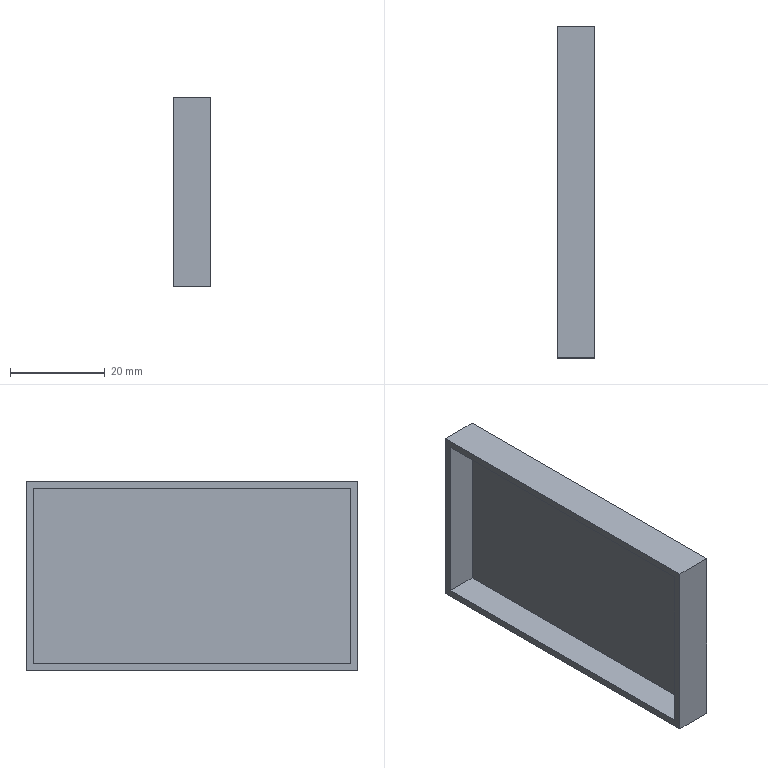Component | SolidWorks | RosinBox-2 | 1 solid | 11 faces | box 8 x 70 x 40 mm | volume 6286 mm3 | plane 11 | material Plain Carbon Steel
build123d program:
from build123d import *

# Parameters (mm, degrees)
SKETCH1_W           = 70
SKETCH1_H           = 40
BOSS_EXTRUDE1_DEPTH = 8
SHELL1_T            = -1.5


with BuildPart() as part:
    # Sketch1 → Boss-Extrude1 (new body)
    with BuildSketch(Plane.XY):
        Rectangle(SKETCH1_W, SKETCH1_H)
    extrude(amount=BOSS_EXTRUDE1_DEPTH)

    # Shell1
    shell1_openings = [part.faces().sort_by_distance(p)[0] for p in [
        (0, 0, 8),
    ]]
    offset(amount=SHELL1_T, openings=shell1_openings, kind=Kind.INTERSECTION)


solid = part.part

# Placed as in the assembly
solid = solid.moved(Location((-806.135, -278.157, 1143.102), (90, -90, 0)))
STEP:
#1=CARTESIAN_POINT('',(-31.738,-9.573,45.791));
#2=VERTEX_POINT('',#1);
#3=CARTESIAN_POINT('',(-31.738,-9.573,44.217));
#4=VERTEX_POINT('',#3);
#5=CARTESIAN_POINT('',(-31.738,-9.573,44.217));
#6=DIRECTION('',(-0.,0.,-1.));
#7=VECTOR('',#6,39.37);
#8=LINE('',#5,#7);
#9=EDGE_CURVE('',#2,#4,#8,.T.);
#10=ORIENTED_EDGE('',*,*,#9,.T.);
#11=CARTESIAN_POINT('',(-32.053,-9.573,44.217));
#12=VERTEX_POINT('',#11);
#13=CARTESIAN_POINT('',(-32.053,-9.573,44.217));
#14=DIRECTION('',(1.,0.,-0.));
#15=VECTOR('',#14,39.37);
#16=LINE('',#13,#15);
#17=EDGE_CURVE('',#12,#4,#16,.T.);
#18=ORIENTED_EDGE('',*,*,#17,.F.);
#19=CARTESIAN_POINT('',(-32.053,-9.573,45.791));
#20=VERTEX_POINT('',#19);
#21=CARTESIAN_POINT('',(-32.053,-9.573,44.217));
#22=DIRECTION('',(-0.,0.,-1.));
#23=VECTOR('',#22,39.37);
#24=LINE('',#21,#23);
#25=EDGE_CURVE('',#20,#12,#24,.T.);
#26=ORIENTED_EDGE('',*,*,#25,.F.);
#27=CARTESIAN_POINT('',(-32.053,-9.573,45.791));
#28=DIRECTION('',(1.,0.,-0.));
#29=VECTOR('',#28,39.37);
#30=LINE('',#27,#29);
#31=EDGE_CURVE('',#20,#2,#30,.T.);
#32=ORIENTED_EDGE('',*,*,#31,.T.);
#33=EDGE_LOOP('',(#10,#18,#26,#32));
#34=FACE_OUTER_BOUND('',#33,.T.);
#35=CARTESIAN_POINT('',(-32.053,-9.573,44.217));
#36=DIRECTION('',(0.,-1.,-0.));
#37=DIRECTION('',(1.,0.,-0.));
#38=AXIS2_PLACEMENT_3D('',#35,#36,#37);
#39=PLANE('',#38);
#40=ADVANCED_FACE('',(#34),#39,.F.);
#41=CARTESIAN_POINT('',(-31.738,-12.329,44.217));
#42=VERTEX_POINT('',#41);
#43=CARTESIAN_POINT('',(-31.738,-12.329,44.217));
#44=DIRECTION('',(0.,-1.,-0.));
#45=VECTOR('',#44,39.37);
#46=LINE('',#43,#45);
#47=EDGE_CURVE('',#4,#42,#46,.T.);
#48=ORIENTED_EDGE('',*,*,#47,.T.);
#49=CARTESIAN_POINT('',(-32.053,-12.329,44.217));
#50=VERTEX_POINT('',#49);
#51=CARTESIAN_POINT('',(-32.053,-12.329,44.217));
#52=DIRECTION('',(1.,0.,-0.));
#53=VECTOR('',#52,39.37);
#54=LINE('',#51,#53);
#55=EDGE_CURVE('',#50,#42,#54,.T.);
#56=ORIENTED_EDGE('',*,*,#55,.F.);
#57=CARTESIAN_POINT('',(-32.053,-12.329,44.217));
#58=DIRECTION('',(0.,-1.,-0.));
#59=VECTOR('',#58,39.37);
#60=LINE('',#57,#59);
#61=EDGE_CURVE('',#12,#50,#60,.T.);
#62=ORIENTED_EDGE('',*,*,#61,.F.);
#63=ORIENTED_EDGE('',*,*,#17,.T.);
#64=EDGE_LOOP('',(#48,#56,#62,#63));
#65=FACE_OUTER_BOUND('',#64,.T.);
#66=CARTESIAN_POINT('',(-32.053,-12.329,44.217));
#67=DIRECTION('',(0.,-0.,1.));
#68=DIRECTION('',(-0.,1.,0.));
#69=AXIS2_PLACEMENT_3D('',#66,#67,#68);
#70=PLANE('',#69);
#71=ADVANCED_FACE('',(#65),#70,.F.);
#72=CARTESIAN_POINT('',(-31.738,-12.329,45.791));
#73=VERTEX_POINT('',#72);
#74=CARTESIAN_POINT('',(-31.738,-12.329,44.217));
#75=DIRECTION('',(0.,-0.,1.));
#76=VECTOR('',#75,39.37);
#77=LINE('',#74,#76);
#78=EDGE_CURVE('',#42,#73,#77,.T.);
#79=ORIENTED_EDGE('',*,*,#78,.T.);
#80=CARTESIAN_POINT('',(-32.053,-12.329,45.791));
#81=VERTEX_POINT('',#80);
#82=CARTESIAN_POINT('',(-32.053,-12.329,45.791));
#83=DIRECTION('',(1.,0.,-0.));
#84=VECTOR('',#83,39.37);
#85=LINE('',#82,#84);
#86=EDGE_CURVE('',#81,#73,#85,.T.);
#87=ORIENTED_EDGE('',*,*,#86,.F.);
#88=CARTESIAN_POINT('',(-32.053,-12.329,44.217));
#89=DIRECTION('',(0.,-0.,1.));
#90=VECTOR('',#89,39.37);
#91=LINE('',#88,#90);
#92=EDGE_CURVE('',#50,#81,#91,.T.);
#93=ORIENTED_EDGE('',*,*,#92,.F.);
#94=ORIENTED_EDGE('',*,*,#55,.T.);
#95=EDGE_LOOP('',(#79,#87,#93,#94));
#96=FACE_OUTER_BOUND('',#95,.T.);
#97=CARTESIAN_POINT('',(-32.053,-12.329,44.217));
#98=DIRECTION('',(-0.,1.,0.));
#99=DIRECTION('',(-1.,-0.,0.));
#100=AXIS2_PLACEMENT_3D('',#97,#98,#99);
#101=PLANE('',#100);
#102=ADVANCED_FACE('',(#96),#101,.F.);
#103=CARTESIAN_POINT('',(-31.738,-12.329,45.791));
#104=DIRECTION('',(-0.,1.,0.));
#105=VECTOR('',#104,39.37);
#106=LINE('',#103,#105);
#107=EDGE_CURVE('',#73,#2,#106,.T.);
#108=ORIENTED_EDGE('',*,*,#107,.T.);
#109=ORIENTED_EDGE('',*,*,#31,.F.);
#110=CARTESIAN_POINT('',(-32.053,-12.329,45.791));
#111=DIRECTION('',(-0.,1.,0.));
#112=VECTOR('',#111,39.37);
#113=LINE('',#110,#112);
#114=EDGE_CURVE('',#81,#20,#113,.T.);
#115=ORIENTED_EDGE('',*,*,#114,.F.);
#116=ORIENTED_EDGE('',*,*,#86,.T.);
#117=EDGE_LOOP('',(#108,#109,#115,#116));
#118=FACE_OUTER_BOUND('',#117,.T.);
#119=CARTESIAN_POINT('',(-32.053,-12.329,45.791));
#120=DIRECTION('',(-0.,0.,-1.));
#121=DIRECTION('',(0.,-1.,-0.));
#122=AXIS2_PLACEMENT_3D('',#119,#120,#121);
#123=PLANE('',#122);
#124=ADVANCED_FACE('',(#118),#123,.F.);
#125=CARTESIAN_POINT('',(-32.053,-9.632,45.732));
#126=VERTEX_POINT('',#125);
#127=CARTESIAN_POINT('',(-32.053,-9.632,44.276));
#128=VERTEX_POINT('',#127);
#129=CARTESIAN_POINT('',(-32.053,-9.632,44.217));
#130=DIRECTION('',(-0.,0.,-1.));
#131=VECTOR('',#130,39.37);
#132=LINE('',#129,#131);
#133=EDGE_CURVE('',#126,#128,#132,.T.);
#134=ORIENTED_EDGE('',*,*,#133,.F.);
#135=CARTESIAN_POINT('',(-32.053,-12.27,45.732));
#136=VERTEX_POINT('',#135);
#137=CARTESIAN_POINT('',(-32.053,-12.329,45.732));
#138=DIRECTION('',(-0.,1.,0.));
#139=VECTOR('',#138,39.37);
#140=LINE('',#137,#139);
#141=EDGE_CURVE('',#136,#126,#140,.T.);
#142=ORIENTED_EDGE('',*,*,#141,.F.);
#143=CARTESIAN_POINT('',(-32.053,-12.27,44.276));
#144=VERTEX_POINT('',#143);
#145=CARTESIAN_POINT('',(-32.053,-12.27,44.217));
#146=DIRECTION('',(0.,-0.,1.));
#147=VECTOR('',#146,39.37);
#148=LINE('',#145,#147);
#149=EDGE_CURVE('',#144,#136,#148,.T.);
#150=ORIENTED_EDGE('',*,*,#149,.F.);
#151=CARTESIAN_POINT('',(-32.053,-12.329,44.276));
#152=DIRECTION('',(0.,-1.,-0.));
#153=VECTOR('',#152,39.37);
#154=LINE('',#151,#153);
#155=EDGE_CURVE('',#128,#144,#154,.T.);
#156=ORIENTED_EDGE('',*,*,#155,.F.);
#157=EDGE_LOOP('',(#134,#142,#150,#156));
#158=FACE_BOUND('',#157,.T.);
#159=ORIENTED_EDGE('',*,*,#25,.T.);
#160=ORIENTED_EDGE('',*,*,#61,.T.);
#161=ORIENTED_EDGE('',*,*,#92,.T.);
#162=ORIENTED_EDGE('',*,*,#114,.T.);
#163=EDGE_LOOP('',(#159,#160,#161,#162));
#164=FACE_OUTER_BOUND('',#163,.T.);
#165=CARTESIAN_POINT('',(-32.053,-10.951,45.004));
#166=DIRECTION('',(-1.,-0.,0.));
#167=DIRECTION('',(0.,-1.,-0.));
#168=AXIS2_PLACEMENT_3D('',#165,#166,#167);
#169=PLANE('',#168);
#170=ADVANCED_FACE('',(#158,#164),#169,.T.);
#171=ORIENTED_EDGE('',*,*,#9,.F.);
#172=ORIENTED_EDGE('',*,*,#107,.F.);
#173=ORIENTED_EDGE('',*,*,#78,.F.);
#174=ORIENTED_EDGE('',*,*,#47,.F.);
#175=EDGE_LOOP('',(#171,#172,#173,#174));
#176=FACE_OUTER_BOUND('',#175,.T.);
#177=CARTESIAN_POINT('',(-31.738,-10.951,45.004));
#178=DIRECTION('',(-1.,-0.,0.));
#179=DIRECTION('',(0.,-1.,-0.));
#180=AXIS2_PLACEMENT_3D('',#177,#178,#179);
#181=PLANE('',#180);
#182=ADVANCED_FACE('',(#176),#181,.F.);
#183=CARTESIAN_POINT('',(-31.797,-9.632,45.732));
#184=VERTEX_POINT('',#183);
#185=CARTESIAN_POINT('',(-31.797,-9.632,44.276));
#186=VERTEX_POINT('',#185);
#187=CARTESIAN_POINT('',(-31.797,-9.632,44.217));
#188=DIRECTION('',(-0.,0.,-1.));
#189=VECTOR('',#188,39.37);
#190=LINE('',#187,#189);
#191=EDGE_CURVE('',#184,#186,#190,.T.);
#192=ORIENTED_EDGE('',*,*,#191,.F.);
#193=CARTESIAN_POINT('',(-32.053,-9.632,45.732));
#194=DIRECTION('',(1.,0.,-0.));
#195=VECTOR('',#194,39.37);
#196=LINE('',#193,#195);
#197=EDGE_CURVE('',#126,#184,#196,.T.);
#198=ORIENTED_EDGE('',*,*,#197,.F.);
#199=ORIENTED_EDGE('',*,*,#133,.T.);
#200=CARTESIAN_POINT('',(-32.053,-9.632,44.276));
#201=DIRECTION('',(1.,0.,-0.));
#202=VECTOR('',#201,39.37);
#203=LINE('',#200,#202);
#204=EDGE_CURVE('',#128,#186,#203,.T.);
#205=ORIENTED_EDGE('',*,*,#204,.T.);
#206=EDGE_LOOP('',(#192,#198,#199,#205));
#207=FACE_OUTER_BOUND('',#206,.T.);
#208=CARTESIAN_POINT('',(-32.053,-9.632,44.217));
#209=DIRECTION('',(0.,-1.,-0.));
#210=DIRECTION('',(1.,0.,-0.));
#211=AXIS2_PLACEMENT_3D('',#208,#209,#210);
#212=PLANE('',#211);
#213=ADVANCED_FACE('',(#207),#212,.T.);
#214=CARTESIAN_POINT('',(-31.797,-12.27,44.276));
#215=VERTEX_POINT('',#214);
#216=CARTESIAN_POINT('',(-31.797,-12.329,44.276));
#217=DIRECTION('',(0.,-1.,-0.));
#218=VECTOR('',#217,39.37);
#219=LINE('',#216,#218);
#220=EDGE_CURVE('',#186,#215,#219,.T.);
#221=ORIENTED_EDGE('',*,*,#220,.F.);
#222=ORIENTED_EDGE('',*,*,#204,.F.);
#223=ORIENTED_EDGE('',*,*,#155,.T.);
#224=CARTESIAN_POINT('',(-32.053,-12.27,44.276));
#225=DIRECTION('',(1.,0.,-0.));
#226=VECTOR('',#225,39.37);
#227=LINE('',#224,#226);
#228=EDGE_CURVE('',#144,#215,#227,.T.);
#229=ORIENTED_EDGE('',*,*,#228,.T.);
#230=EDGE_LOOP('',(#221,#222,#223,#229));
#231=FACE_OUTER_BOUND('',#230,.T.);
#232=CARTESIAN_POINT('',(-32.053,-12.329,44.276));
#233=DIRECTION('',(0.,-0.,1.));
#234=DIRECTION('',(-0.,1.,0.));
#235=AXIS2_PLACEMENT_3D('',#232,#233,#234);
#236=PLANE('',#235);
#237=ADVANCED_FACE('',(#231),#236,.T.);
#238=CARTESIAN_POINT('',(-31.797,-12.27,45.732));
#239=VERTEX_POINT('',#238);
#240=CARTESIAN_POINT('',(-31.797,-12.27,44.217));
#241=DIRECTION('',(0.,-0.,1.));
#242=VECTOR('',#241,39.37);
#243=LINE('',#240,#242);
#244=EDGE_CURVE('',#215,#239,#243,.T.);
#245=ORIENTED_EDGE('',*,*,#244,.F.);
#246=ORIENTED_EDGE('',*,*,#228,.F.);
#247=ORIENTED_EDGE('',*,*,#149,.T.);
#248=CARTESIAN_POINT('',(-32.053,-12.27,45.732));
#249=DIRECTION('',(1.,0.,-0.));
#250=VECTOR('',#249,39.37);
#251=LINE('',#248,#250);
#252=EDGE_CURVE('',#136,#239,#251,.T.);
#253=ORIENTED_EDGE('',*,*,#252,.T.);
#254=EDGE_LOOP('',(#245,#246,#247,#253));
#255=FACE_OUTER_BOUND('',#254,.T.);
#256=CARTESIAN_POINT('',(-32.053,-12.27,44.217));
#257=DIRECTION('',(-0.,1.,0.));
#258=DIRECTION('',(-1.,-0.,0.));
#259=AXIS2_PLACEMENT_3D('',#256,#257,#258);
#260=PLANE('',#259);
#261=ADVANCED_FACE('',(#255),#260,.T.);
#262=CARTESIAN_POINT('',(-31.797,-12.329,45.732));
#263=DIRECTION('',(-0.,1.,0.));
#264=VECTOR('',#263,39.37);
#265=LINE('',#262,#264);
#266=EDGE_CURVE('',#239,#184,#265,.T.);
#267=ORIENTED_EDGE('',*,*,#266,.F.);
#268=ORIENTED_EDGE('',*,*,#252,.F.);
#269=ORIENTED_EDGE('',*,*,#141,.T.);
#270=ORIENTED_EDGE('',*,*,#197,.T.);
#271=EDGE_LOOP('',(#267,#268,#269,#270));
#272=FACE_OUTER_BOUND('',#271,.T.);
#273=CARTESIAN_POINT('',(-32.053,-12.329,45.732));
#274=DIRECTION('',(-0.,0.,-1.));
#275=DIRECTION('',(0.,-1.,-0.));
#276=AXIS2_PLACEMENT_3D('',#273,#274,#275);
#277=PLANE('',#276);
#278=ADVANCED_FACE('',(#272),#277,.T.);
#279=ORIENTED_EDGE('',*,*,#191,.T.);
#280=ORIENTED_EDGE('',*,*,#220,.T.);
#281=ORIENTED_EDGE('',*,*,#244,.T.);
#282=ORIENTED_EDGE('',*,*,#266,.T.);
#283=EDGE_LOOP('',(#279,#280,#281,#282));
#284=FACE_OUTER_BOUND('',#283,.T.);
#285=CARTESIAN_POINT('',(-31.797,-10.951,45.004));
#286=DIRECTION('',(-1.,-0.,0.));
#287=DIRECTION('',(0.,-1.,-0.));
#288=AXIS2_PLACEMENT_3D('',#285,#286,#287);
#289=PLANE('',#288);
#290=ADVANCED_FACE('',(#284),#289,.T.);
#291=CLOSED_SHELL('',(#40,#71,#102,#124,#170,#182,#213,#237,#261,#278,#290));
#292=MANIFOLD_SOLID_BREP('',#291);
#293=CARTESIAN_POINT('',(0.,0.,0.));
#294=DIRECTION('',(0.,0.,1.));
#295=DIRECTION('',(1.,0.,0.));
#296=AXIS2_PLACEMENT_3D('',#293,#294,#295);
#297=(LENGTH_UNIT()NAMED_UNIT(*)SI_UNIT($,.METRE.));
#298=LENGTH_MEASURE_WITH_UNIT(LENGTH_MEASURE(0.0254),#297);
#299=DIMENSIONAL_EXPONENTS(1.,0.,0.,0.,0.,0.,0.);
#300=(CONVERSION_BASED_UNIT('',#298)LENGTH_UNIT()NAMED_UNIT(#299));
#301=UNCERTAINTY_MEASURE_WITH_UNIT(LENGTH_MEASURE(0.00001),#300,'','');
#302=(NAMED_UNIT(*)PLANE_ANGLE_UNIT()SI_UNIT($,.RADIAN.));
#303=(NAMED_UNIT(*)SI_UNIT($,.STERADIAN.)SOLID_ANGLE_UNIT());
#304=(GEOMETRIC_REPRESENTATION_CONTEXT(3)GLOBAL_UNCERTAINTY_ASSIGNED_CONTEXT((#301))GLOBAL_UNIT_ASSIGNED_CONTEXT((#300,#302,#303))REPRESENTATION_CONTEXT('',''));
#305=ADVANCED_BREP_SHAPE_REPRESENTATION('',(#292,#296),#304);
#306=COLOUR_RGB('',0.7922,0.8196,0.9333);
#307=FILL_AREA_STYLE_COLOUR('',#306);
#308=FILL_AREA_STYLE('',(#307));
#309=SURFACE_STYLE_FILL_AREA(#308);
#310=SURFACE_SIDE_STYLE('',(#309));
#311=SURFACE_STYLE_USAGE(.BOTH.,#310);
#312=PRESENTATION_STYLE_ASSIGNMENT((#311));
#313=STYLED_ITEM('',(#312),#292);
#314=PRESENTATION_LAYER_ASSIGNMENT('','',(#313));
#315=(LENGTH_UNIT()NAMED_UNIT(*)SI_UNIT($,.METRE.));
#316=LENGTH_MEASURE_WITH_UNIT(LENGTH_MEASURE(0.0254),#315);
#317=DIMENSIONAL_EXPONENTS(1.,0.,0.,0.,0.,0.,0.);
#318=(CONVERSION_BASED_UNIT('',#316)LENGTH_UNIT()NAMED_UNIT(#317));
#319=UNCERTAINTY_MEASURE_WITH_UNIT(LENGTH_MEASURE(0.00001),#318,'','');
#320=(NAMED_UNIT(*)PLANE_ANGLE_UNIT()SI_UNIT($,.RADIAN.));
#321=(NAMED_UNIT(*)SI_UNIT($,.STERADIAN.)SOLID_ANGLE_UNIT());
#322=(GEOMETRIC_REPRESENTATION_CONTEXT(3)GLOBAL_UNCERTAINTY_ASSIGNED_CONTEXT((#319))GLOBAL_UNIT_ASSIGNED_CONTEXT((#318,#320,#321))REPRESENTATION_CONTEXT('',''));
#323=MECHANICAL_DESIGN_GEOMETRIC_PRESENTATION_REPRESENTATION('',(#313),#322);